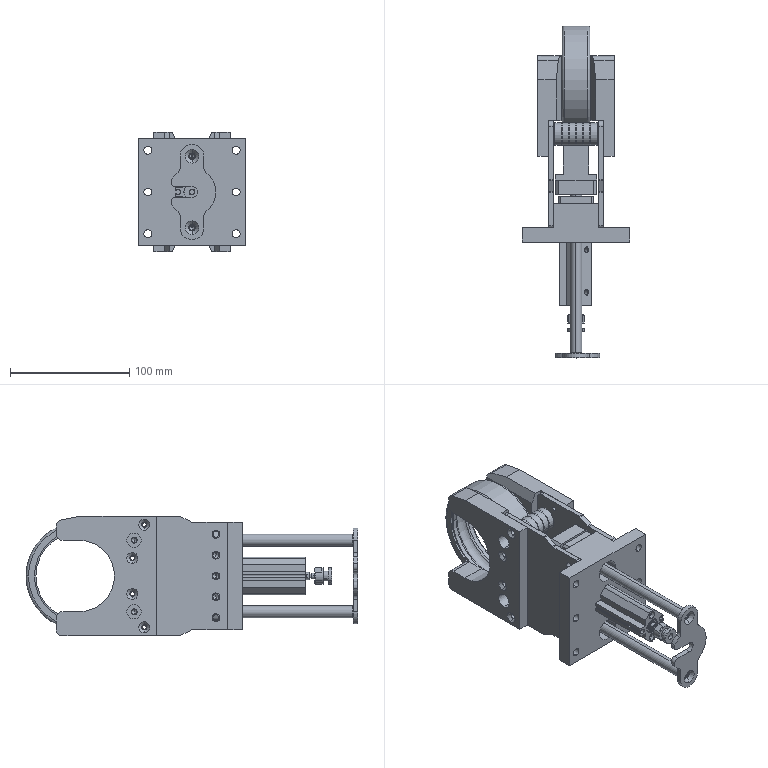Assembly | SolidWorks | mm | 28 component files | 29 solids | 1920 faces | box 90 x 278.12 x 100 mm | volume 556366 mm3 | cylinder 652 | cone 607 | plane 359 | torus 302 | commonest cylinder face diameters 11.5 x48 15.5 x48 11.284 x48 11 x48 16.6 x48 10.6 x48 8 x36 3.3 x32
Bill of materials:
6308-OuterRing | 1 | AISI 304 | Thin-walled short cylindrical ring with rounded outer edges and shallow internal circumferential steps/grooves.
BAF698ZZ-SUS.stp | 12 | AISI 304 | Annular body resembling a shielded radial ball bearing: outer ring, recessed annular face/shield, and inner ring with central bore.
BlankingGuidePost-136 | 2 | 45 | Long slender thin-walled tube with plain square ends and a small concentric bore.
cylinder_cdq2b12-25dm.stp | 1 |  | Compact prismatic actuator-like body with a projecting stepped cylindrical rod at one end, an irregular polygonal end face with through holes and open slots, longitudinal grooves along the sides, and transverse holes on one flat face.
LME13-d10.stp | 2 |  | Flanged cylindrical sleeve/bushing: square flange with chamfered corners and four corner through holes, with a cylindrical boss carrying a central through bore.
MHF04-D8-L38.stp | 2 |  | Cylindrical tube/spacer with chamfered ends and a concentric bore.
QX1-12-V-BracketBase | 1 | 6061 Alloy | Rectangular plate with a raised rectangular block/tab on one edge, two large through holes, six smaller corner/edge through holes, and small central holes.
QX1-13-BJV-Bracket | 1 | Q235 | Thin flat plate with one rounded corner, a stepped/angled offset along two opposite edges, a column of five larger holes along one side and a column of six alternating larger and smaller holes along the opposite side.
QX1-14-BJV-BracketB | 1 | Q235 | Thin flat plate with one rounded corner, angled steps in the outline, a column of five larger holes on one side and an alternating pattern of larger and smaller holes on the opposite side.
QX1-15-PusherSlider | 1 | PA Type 6 | Bracket-like block: a rectangular plate with chamfered corners and two counterbored/stepped holes, joined to a projecting tapered (trapezoidal-profile) web or lug, with a small notch/step on one face.
QX1-16-BJPusherCylinderConnectionBlock | 1 | Q235 | Thin flat hook/latch-like plate with rounded ends, two countersunk mounting holes, and a side slot with a rounded inner end forming a hook profile.
QX1-17-V-BracketSidePlate | 1 | PA Type 6 | Plate with a large semicircular-ended U-shaped cutout open on one edge, a column of holes along the opposite edge (four countersunk smaller holes and two larger plain holes), and a stepped/chamfered edge profile.
QX1-46-V-BracketSidePlate | 1 | PA Type 6 | Plate-like bracket. One side is a thicker rectangular strip with a row of through holes. The other side is a thinner fork (C-shape) with two arms around a large rounded, roughly semicircular cutout. The arm ends have rounded corners and the upper arm has a sloped or chamfered top surface.
WHC61-M5-0.8-L4.stp | 1 | AISI 304 | Spool-shaped bushing that is round about its axis, with a central through bore. It has two outer cylindrical sections of roughly equal diameter joined by a smaller-diameter neck, which forms a groove between them. One outer section is longer than the other and has a flat face on part of its outer surface. All outer edges have small chamfers.
Mates:
1. distance | QX1-13-BJV-Bracket-1 face at (19, 102, 0) dir (-1, 0, 0) | BAF698ZZ-SUS.stp-1 face at (18, 85.433, -29.585) dir (1, 0, 0)
2. concentric | QX1-13-BJV-Bracket-1 face at (23, 90.617, -30) dir (1, 0, 0) r 2.55 | BAF698ZZ-SUS.stp-1 face at (12.3, 90.617, -30) dir (1, 0, 0) r 4
3. distance | QX1-13-BJV-Bracket-1 face at (19, 102, 0) dir (-1, 0, 0) | BAF698ZZ-SUS.stp-2 face at (18, 85.535, 28.898) dir (1, 0, 0)
4. concentric | QX1-13-BJV-Bracket-1 face at (23, 90.617, 30) dir (1, 0, 0) r 2.55 | BAF698ZZ-SUS.stp-2 face at (12.3, 90.617, 30) dir (1, 0, 0) r 4
5. concentric | BAF698ZZ-SUS.stp-8 face at (-5.7, 90.617, -30) dir (1, 0, 0) r 9.5 | QX1-14-BJV-BracketB-1 face at (-19, 90.617, -30) dir (1, 0, 0) r 2.55
6. concentric | BAF698ZZ-SUS.stp-5 face at (-5.7, 90.617, 30) dir (1, 0, 0) r 4 | QX1-14-BJV-BracketB-1 face at (-19, 90.617, 30) dir (1, 0, 0) r 2.55
7. distance | QX1-13-BJV-Bracket-1 face at (19, 102, 0) dir (-1, 0, 0) | QX1-14-BJV-BracketB-1 face at (-19, 102, 0) dir (1, 0, 0)
8. coincident | QX1-14-BJV-BracketB-1 face at (-19, 102, 0) dir (1, 0, 0) | QX1-12-V-BracketBase-1 face at (-19, 32, 45) dir (-1, 0, 0)
9. coincident | QX1-13-BJV-Bracket-1 face at (23, 12, -45) dir (0, -1, 0) | QX1-12-V-BracketBase-1 face at (45, 12, 45) dir (0, 1, 0)
10. coincident | QX1-14-BJV-BracketB-1 face at (-19, 12, -45) dir (0, 0, -1) | QX1-12-V-BracketBase-1 face at (0, 0, -45) dir (0, 0, -1)
11. parallel | QX1-12-V-BracketBase-1 face at (19, 32, 45) dir (0, 1, 0) | QX1-15-PusherSlider-1 face at (-17.5, 40, 19.5) dir (0, -1, 0)
12. distance | QX1-15-PusherSlider-1 face at (-17.5, 40, -19.5) dir (0, 0, -1) | QX1-13-BJV-Bracket-1 face at (23, 52, -50) dir (0, 0, -1)
13. coordinate | QX1-12-V-BracketBase-1 sketch point at (0, 0, 0) dir (1, 0, 0) | assembly sketch point at (0, 0, 0) dir (1, 0, 0)
14. coincident | QX1-12-V-BracketBase-1 face at (19, 32, 45) dir (0, 1, 0) | LME13-d10.stp-2 face at (0, 32, 30) dir (0, -1, 0)
15. coincident | QX1-12-V-BracketBase-1 face at (19, 32, 45) dir (0, 1, 0) | LME13-d10.stp-1 face at (0, 32, -30) dir (0, -1, 0)
16. concentric | QX1-12-V-BracketBase-1 face at (0, 32, 30) dir (0, -1, 0) r 9.5 | LME13-d10.stp-2 face at (0, 38, 30) dir (0, -1, 0) r 9.5
17. concentric | QX1-12-V-BracketBase-1 face at (0, 32, -30) dir (0, -1, 0) r 9.5 | LME13-d10.stp-1 face at (0, 38, -30) dir (0, -1, 0) r 5
18. parallel | LME13-d10.stp-1 face at (-15, 32, -16.771) dir (-1, 0, 0) | LME13-d10.stp-2 face at (-15, 32, 43.229) dir (-1, 0, 0)
19. parallel | QX1-12-V-BracketBase-1 face at (-19, 32, 45) dir (-1, 0, 0) | LME13-d10.stp-2 face at (-15, 32, 43.229) dir (-1, 0, 0)
20. distance | QX1-15-PusherSlider-1 face at (-17.5, 40, 19.5) dir (0, -1, 0) | QX1-12-V-BracketBase-1 face at (19, 32, 45) dir (0, 1, 0)
21. concentric | LME13-d10.stp-1 face at (0, 38, -30) dir (0, -1, 0) r 5 | BlankingGuidePost-136-1 face at (0, -93, -30) dir (0, 1, 0) r 5
22. coincident | QX1-15-PusherSlider-1 face at (0, 43, -30) dir (0, -1, 0) | BlankingGuidePost-136-1 face at (0, 43, -30) dir (0, 1, 0)
23. width | QX1-15-PusherSlider-1 face at (17.5, 40, -19.5) dir (1, 0, 0) | QX1-15-PusherSlider-1 face at (-17.5, 40, -19.5) dir (-1, 0, 0) | QX1-12-V-BracketBase-1 face at (-45, 12, 45) dir (-1, 0, 0) | QX1-12-V-BracketBase-1 face at (45, 0, 45) dir (1, 0, 0)
24. concentric | QX1-15-PusherSlider-1 face at (0, 43, 30) dir (0, -1, 0) r 5 | BlankingGuidePost-136-2 face at (0, -93, 30) dir (0, 1, 0) r 5
25. coincident | BlankingGuidePost-136-1 face at (0, -93, -30) dir (0, -1, 0) | BlankingGuidePost-136-2 face at (0, -93, 30) dir (0, -1, 0)
26. coincident | BlankingGuidePost-136-2 face at (0, -93, 30) dir (0, -1, 0) | QX1-16-BJPusherCylinderConnectionBlock-1 face at (0, -93, 30) dir (0, 1, 0)
27. concentric | BlankingGuidePost-136-2 face at (0, -93, 30) dir (0, 1, 0) r 5 | QX1-16-BJPusherCylinderConnectionBlock-1 face at (0, -97, 30) dir (0, -1, 0) r 2.75
28. coincident | QX1-13-BJV-Bracket-1 face at (19, 102, 0) dir (-1, 0, 0) | MHF04-D8-L38.stp-1 face at (19, 94.117, -30) dir (1, 0, 0)
29. concentric | BAF698ZZ-SUS.stp-1 face at (12.3, 90.617, -30) dir (1, 0, 0) r 9.5 | MHF04-D8-L38.stp-1 face at (19, 90.617, -30) dir (-1, 0, 0) r 4
30. coincident | QX1-14-BJV-BracketB-1 face at (-19, 102, 0) dir (1, 0, 0) | MHF04-D8-L38.stp-2 face at (-19, 93.117, 30) dir (-1, 0, 0)
31. concentric | BAF698ZZ-SUS.stp-14 face at (-17.7, 90.617, 30) dir (1, 0, 0) r 9.5 | MHF04-D8-L38.stp-2 face at (19, 90.617, 30) dir (-1, 0, 0) r 4
32. coincident | QX1-13-BJV-Bracket-1 face at (23, 102, 0) dir (1, 0, 0) | QX1-17-V-BracketSidePlate-2 face at (23, 102, 0) dir (-1, 0, 0)
33. coincident | QX1-13-BJV-Bracket-1 face at (23, 102, -50) dir (0, 1, 0) | QX1-17-V-BracketSidePlate-2 face at (24, 102, 50) dir (0, -1, 0)
34. coincident | QX1-13-BJV-Bracket-1 face at (23, 52, -50) dir (0, 0, -1) | QX1-17-V-BracketSidePlate-2 face at (32, 132, -50) dir (0, 0, -1)
35. width | 6308-OuterRing-1 face at (-11.55, 136.117, 0) dir (-1, 0, 0) | 6308-OuterRing-1 face at (11.55, 136.117, 0) dir (1, 0, 0) | QX1-13-BJV-Bracket-1 face at (23, 102, 0) dir (1, 0, 0) | QX1-14-BJV-BracketB-1 face at (-23, 102, 0) dir (-1, 0, 0)
36. coincident | 6308-OuterRing-1 plane at (0, 136.117, 0) dir (0, 0, -1) | assembly plane at (0, 0, 0) dir (0, 0, 1)
37. tangent | BAF698ZZ-SUS.stp-8 face at (-5.7, 90.617, -30) dir (1, 0, 0) r 9.5 | 6308-OuterRing-1 face at (11.55, 136.117, 0) dir (-1, 0, 0) r 45
38. coincident | QX1-12-V-BracketBase-1 face at (-45, 0, 45) dir (0, -1, 0) | cylinder_cdq2b12-25dm.stp-1 face at (0.2283, 0, 0) dir (0, 1, 0)
39. concentric | WHC61-M5-0.8-L4.stp-1 face at (0, -25, 0) dir (0, -1, 0) r 6.75 | cylinder_cdq2b12-25dm.stp-1 face at (0, -62.5, 0) dir (0, 1, 0) r 2.5
40. distance | WHC61-M5-0.8-L4.stp-1 face at (3.577, -61, -5.487) dir (0, 1, 0) | cylinder_cdq2b12-25dm.stp-1 face at (-1.034, -67, 0) dir (0, -1, 0)
41. concentric | QX1-12-V-BracketBase-1 face at (0, 0, 11) dir (0, -1, 0) r 1.25 | cylinder_cdq2b12-25dm.stp-1 face at (0, -51.75, 11) dir (0, 1, 0) r 3.25
42. concentric | QX1-12-V-BracketBase-1 face at (0, 0, -11) dir (0, -1, 0) r 1.25 | cylinder_cdq2b12-25dm.stp-1 face at (0, -26.5, -11) dir (0, 1, 0) r 1.75
43. parallel | QX1-12-V-BracketBase-1 face at (45, 0, 45) dir (1, 0, 0) | QX1-16-BJPusherCylinderConnectionBlock-1 face at (10, -97, 30) dir (1, 0, 0)